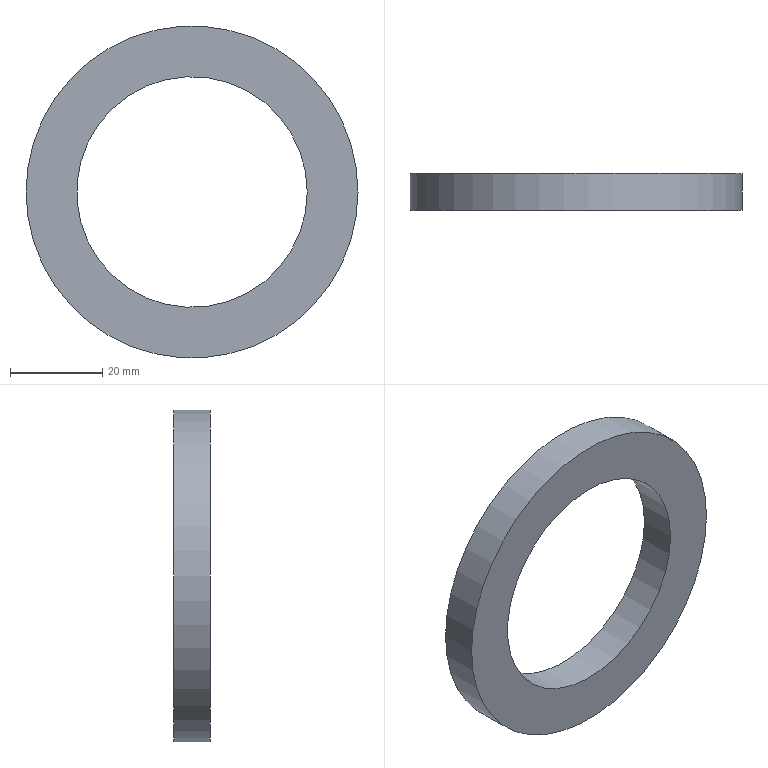Component | NX | OIL_SEAL_72X50X8_4 | 1 solid | 4 faces | box 72 x 8 x 72 mm | volume 16864 mm3 | cylinder 2 | plane 2 | commonest cylinder face diameters 72 x1 50 x1
STEP:
#1=CARTESIAN_POINT('',(0.,0.,0.));
#2=DIRECTION('',(0.,0.,1.));
#3=DIRECTION('',(1.,0.,0.));
#4=AXIS2_PLACEMENT_3D('',#1,#2,#3);
#5=CARTESIAN_POINT('',(33.,129.,-3.));
#6=VERTEX_POINT('',#5);
#7=CARTESIAN_POINT('',(-3.,129.,-3.));
#8=DIRECTION('',(0.,-1.,0.));
#9=DIRECTION('',(1.,0.,0.));
#10=AXIS2_PLACEMENT_3D('',#7,#8,#9);
#11=CIRCLE('',#10,36.);
#12=CARTESIAN_POINT('',(-3.,129.,-3.));
#13=DIRECTION('',(0.,1.,0.));
#14=DIRECTION('',(-1.,0.,0.));
#15=AXIS2_PLACEMENT_3D('',#12,#13,#14);
#16=CYLINDRICAL_SURFACE('',#15,36.);
#17=CARTESIAN_POINT('',(9.425,0.));
#18=DIRECTION('',(-1.,0.));
#19=VECTOR('',#18,1.);
#20=LINE('',#17,#19);
#21=(GEOMETRIC_REPRESENTATION_CONTEXT(2)PARAMETRIC_REPRESENTATION_CONTEXT()REPRESENTATION_CONTEXT('',''));
#22=DEFINITIONAL_REPRESENTATION('',(#20),#21);
#23=PCURVE('',#16,#22);
#24=CARTESIAN_POINT('',(-3.,129.,-3.));
#25=DIRECTION('',(0.,-1.,0.));
#26=DIRECTION('',(1.,0.,0.));
#27=AXIS2_PLACEMENT_3D('',#24,#25,#26);
#28=PLANE('',#27);
#29=CARTESIAN_POINT('',(0.,0.));
#30=DIRECTION('',(1.,0.));
#31=AXIS2_PLACEMENT_2D('',#29,#30);
#32=CIRCLE('',#31,36.);
#33=(GEOMETRIC_REPRESENTATION_CONTEXT(2)PARAMETRIC_REPRESENTATION_CONTEXT()REPRESENTATION_CONTEXT('',''));
#34=DEFINITIONAL_REPRESENTATION('',(#32),#33);
#35=PCURVE('',#28,#34);
#36=SURFACE_CURVE('',#11,(#23,#35),.PCURVE_S1.);
#37=EDGE_CURVE('',#6,#6,#36,.T.);
#38=ORIENTED_EDGE('',*,*,#37,.F.);
#39=CARTESIAN_POINT('',(33.,137.,-3.));
#40=VERTEX_POINT('',#39);
#41=CARTESIAN_POINT('',(33.,129.,-3.));
#42=CARTESIAN_POINT('',(33.,137.,-3.));
#43=B_SPLINE_CURVE_WITH_KNOTS('',1,(#41,#42),.UNSPECIFIED.,.F.,.F.,(2,2),(0.,8.),.PIECEWISE_BEZIER_KNOTS.);
#44=CARTESIAN_POINT('',(9.425,0.));
#45=DIRECTION('',(0.,1.));
#46=VECTOR('',#45,1.);
#47=LINE('',#44,#46);
#48=(GEOMETRIC_REPRESENTATION_CONTEXT(2)PARAMETRIC_REPRESENTATION_CONTEXT()REPRESENTATION_CONTEXT('',''));
#49=DEFINITIONAL_REPRESENTATION('',(#47),#48);
#50=PCURVE('',#16,#49);
#51=CARTESIAN_POINT('',(3.142,0.));
#52=DIRECTION('',(0.,1.));
#53=VECTOR('',#52,1.);
#54=LINE('',#51,#53);
#55=(GEOMETRIC_REPRESENTATION_CONTEXT(2)PARAMETRIC_REPRESENTATION_CONTEXT()REPRESENTATION_CONTEXT('',''));
#56=DEFINITIONAL_REPRESENTATION('',(#54),#55);
#57=PCURVE('',#16,#56);
#58=SEAM_CURVE('',#43,(#50,#57),.PCURVE_S1.);
#59=EDGE_CURVE('',#6,#40,#58,.T.);
#60=ORIENTED_EDGE('',*,*,#59,.T.);
#61=CARTESIAN_POINT('',(-3.,137.,-3.));
#62=DIRECTION('',(0.,-1.,0.));
#63=DIRECTION('',(1.,0.,0.));
#64=AXIS2_PLACEMENT_3D('',#61,#62,#63);
#65=CIRCLE('',#64,36.);
#66=CARTESIAN_POINT('',(9.425,8.));
#67=DIRECTION('',(-1.,0.));
#68=VECTOR('',#67,1.);
#69=LINE('',#66,#68);
#70=(GEOMETRIC_REPRESENTATION_CONTEXT(2)PARAMETRIC_REPRESENTATION_CONTEXT()REPRESENTATION_CONTEXT('',''));
#71=DEFINITIONAL_REPRESENTATION('',(#69),#70);
#72=PCURVE('',#16,#71);
#73=CARTESIAN_POINT('',(-3.,137.,-3.));
#74=DIRECTION('',(0.,-1.,0.));
#75=DIRECTION('',(1.,0.,0.));
#76=AXIS2_PLACEMENT_3D('',#73,#74,#75);
#77=PLANE('',#76);
#78=CARTESIAN_POINT('',(0.,0.));
#79=DIRECTION('',(1.,0.));
#80=AXIS2_PLACEMENT_2D('',#78,#79);
#81=CIRCLE('',#80,36.);
#82=(GEOMETRIC_REPRESENTATION_CONTEXT(2)PARAMETRIC_REPRESENTATION_CONTEXT()REPRESENTATION_CONTEXT('',''));
#83=DEFINITIONAL_REPRESENTATION('',(#81),#82);
#84=PCURVE('',#77,#83);
#85=SURFACE_CURVE('',#65,(#72,#84),.PCURVE_S1.);
#86=EDGE_CURVE('',#40,#40,#85,.T.);
#87=ORIENTED_EDGE('',*,*,#86,.T.);
#88=ORIENTED_EDGE('',*,*,#59,.F.);
#89=EDGE_LOOP('',(#38,#60,#87,#88));
#90=FACE_BOUND('',#89,.T.);
#91=ADVANCED_FACE('',(#90),#16,.T.);
#92=CARTESIAN_POINT('',(22.,129.,-3.));
#93=VERTEX_POINT('',#92);
#94=CARTESIAN_POINT('',(-3.,129.,-3.));
#95=DIRECTION('',(0.,-1.,0.));
#96=DIRECTION('',(1.,0.,0.));
#97=AXIS2_PLACEMENT_3D('',#94,#95,#96);
#98=CIRCLE('',#97,25.);
#99=CARTESIAN_POINT('',(-3.,129.,-3.));
#100=DIRECTION('',(0.,1.,0.));
#101=DIRECTION('',(-1.,0.,0.));
#102=AXIS2_PLACEMENT_3D('',#99,#100,#101);
#103=CYLINDRICAL_SURFACE('',#102,25.);
#104=CARTESIAN_POINT('',(9.425,0.));
#105=DIRECTION('',(-1.,0.));
#106=VECTOR('',#105,1.);
#107=LINE('',#104,#106);
#108=(GEOMETRIC_REPRESENTATION_CONTEXT(2)PARAMETRIC_REPRESENTATION_CONTEXT()REPRESENTATION_CONTEXT('',''));
#109=DEFINITIONAL_REPRESENTATION('',(#107),#108);
#110=PCURVE('',#103,#109);
#111=CARTESIAN_POINT('',(0.,0.));
#112=DIRECTION('',(1.,0.));
#113=AXIS2_PLACEMENT_2D('',#111,#112);
#114=CIRCLE('',#113,25.);
#115=(GEOMETRIC_REPRESENTATION_CONTEXT(2)PARAMETRIC_REPRESENTATION_CONTEXT()REPRESENTATION_CONTEXT('',''));
#116=DEFINITIONAL_REPRESENTATION('',(#114),#115);
#117=PCURVE('',#28,#116);
#118=SURFACE_CURVE('',#98,(#110,#117),.PCURVE_S1.);
#119=EDGE_CURVE('',#93,#93,#118,.T.);
#120=ORIENTED_EDGE('',*,*,#119,.F.);
#121=CARTESIAN_POINT('',(22.,137.,-3.));
#122=VERTEX_POINT('',#121);
#123=CARTESIAN_POINT('',(22.,129.,-3.));
#124=CARTESIAN_POINT('',(22.,137.,-3.));
#125=B_SPLINE_CURVE_WITH_KNOTS('',1,(#123,#124),.UNSPECIFIED.,.F.,.F.,(2,2),(0.,8.),.PIECEWISE_BEZIER_KNOTS.);
#126=CARTESIAN_POINT('',(9.425,0.));
#127=DIRECTION('',(0.,1.));
#128=VECTOR('',#127,1.);
#129=LINE('',#126,#128);
#130=(GEOMETRIC_REPRESENTATION_CONTEXT(2)PARAMETRIC_REPRESENTATION_CONTEXT()REPRESENTATION_CONTEXT('',''));
#131=DEFINITIONAL_REPRESENTATION('',(#129),#130);
#132=PCURVE('',#103,#131);
#133=CARTESIAN_POINT('',(3.142,0.));
#134=DIRECTION('',(0.,1.));
#135=VECTOR('',#134,1.);
#136=LINE('',#133,#135);
#137=(GEOMETRIC_REPRESENTATION_CONTEXT(2)PARAMETRIC_REPRESENTATION_CONTEXT()REPRESENTATION_CONTEXT('',''));
#138=DEFINITIONAL_REPRESENTATION('',(#136),#137);
#139=PCURVE('',#103,#138);
#140=SEAM_CURVE('',#125,(#132,#139),.PCURVE_S1.);
#141=EDGE_CURVE('',#93,#122,#140,.T.);
#142=ORIENTED_EDGE('',*,*,#141,.T.);
#143=CARTESIAN_POINT('',(-3.,137.,-3.));
#144=DIRECTION('',(0.,-1.,0.));
#145=DIRECTION('',(1.,0.,0.));
#146=AXIS2_PLACEMENT_3D('',#143,#144,#145);
#147=CIRCLE('',#146,25.);
#148=CARTESIAN_POINT('',(9.425,8.));
#149=DIRECTION('',(-1.,0.));
#150=VECTOR('',#149,1.);
#151=LINE('',#148,#150);
#152=(GEOMETRIC_REPRESENTATION_CONTEXT(2)PARAMETRIC_REPRESENTATION_CONTEXT()REPRESENTATION_CONTEXT('',''));
#153=DEFINITIONAL_REPRESENTATION('',(#151),#152);
#154=PCURVE('',#103,#153);
#155=CARTESIAN_POINT('',(0.,0.));
#156=DIRECTION('',(1.,0.));
#157=AXIS2_PLACEMENT_2D('',#155,#156);
#158=CIRCLE('',#157,25.);
#159=(GEOMETRIC_REPRESENTATION_CONTEXT(2)PARAMETRIC_REPRESENTATION_CONTEXT()REPRESENTATION_CONTEXT('',''));
#160=DEFINITIONAL_REPRESENTATION('',(#158),#159);
#161=PCURVE('',#77,#160);
#162=SURFACE_CURVE('',#147,(#154,#161),.PCURVE_S1.);
#163=EDGE_CURVE('',#122,#122,#162,.T.);
#164=ORIENTED_EDGE('',*,*,#163,.T.);
#165=ORIENTED_EDGE('',*,*,#141,.F.);
#166=EDGE_LOOP('',(#120,#142,#164,#165));
#167=FACE_BOUND('',#166,.F.);
#168=ADVANCED_FACE('',(#167),#103,.F.);
#169=ORIENTED_EDGE('',*,*,#37,.T.);
#170=EDGE_LOOP('',(#169));
#171=FACE_BOUND('',#170,.T.);
#172=ORIENTED_EDGE('',*,*,#119,.F.);
#173=EDGE_LOOP('',(#172));
#174=FACE_BOUND('',#173,.T.);
#175=ADVANCED_FACE('',(#171,#174),#28,.T.);
#176=ORIENTED_EDGE('',*,*,#86,.F.);
#177=EDGE_LOOP('',(#176));
#178=FACE_BOUND('',#177,.T.);
#179=ORIENTED_EDGE('',*,*,#163,.T.);
#180=EDGE_LOOP('',(#179));
#181=FACE_BOUND('',#180,.T.);
#182=ADVANCED_FACE('',(#178,#181),#77,.F.);
#183=CLOSED_SHELL('',(#91,#168,#175,#182));
#184=MANIFOLD_SOLID_BREP('',#183);
#185=(LENGTH_UNIT()NAMED_UNIT(*)SI_UNIT(.MILLI.,.METRE.));
#186=UNCERTAINTY_MEASURE_WITH_UNIT(LENGTH_MEASURE(0.00001),#185,'','');
#187=(NAMED_UNIT(*)PLANE_ANGLE_UNIT()SI_UNIT($,.RADIAN.));
#188=(NAMED_UNIT(*)SI_UNIT($,.STERADIAN.)SOLID_ANGLE_UNIT());
#189=(GEOMETRIC_REPRESENTATION_CONTEXT(3)GLOBAL_UNCERTAINTY_ASSIGNED_CONTEXT((#186))GLOBAL_UNIT_ASSIGNED_CONTEXT((#185,#187,#188))REPRESENTATION_CONTEXT('',''));
#190=ADVANCED_BREP_SHAPE_REPRESENTATION('',(#4,#184),#189);